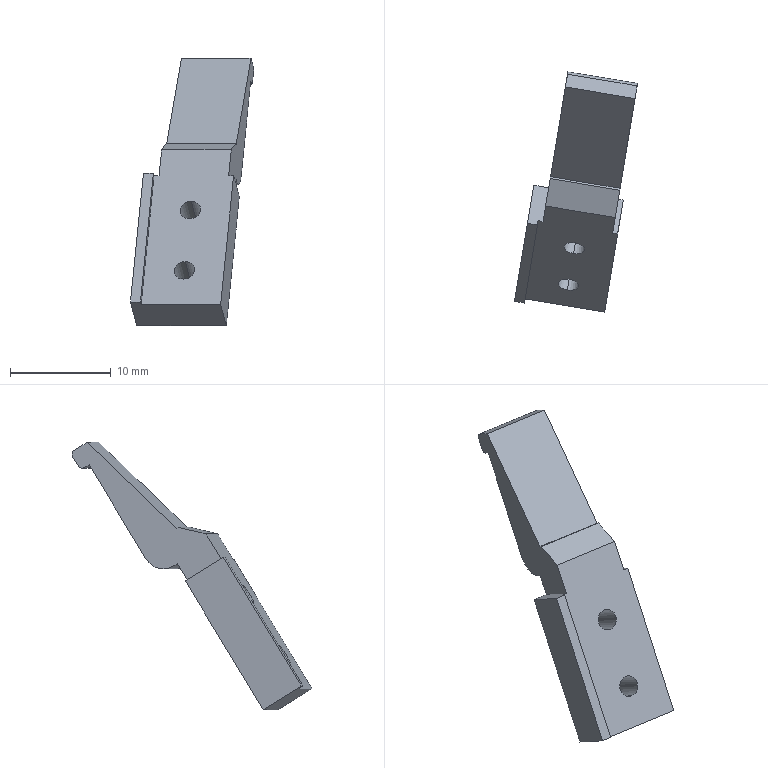Component | SolidWorks | 14AC-24-1-001-1 | 1 solid | 26 faces | box 12.21 x 23.8 x 26.53 mm | volume 925 mm3 | plane 19 | cylinder 7 | commonest cylinder face diameters 2.05 x4 1 x2 4 x1
build123d program:
from build123d import *

# Parameters (mm, degrees)
SKETCH1_W           = 9
SKETCH1_H           = 32
BOSS_EXTRUDE1_DEPTH = 7.45
SKETCH3_W           = 3.45
SKETCH3_H           = 17
CUT_EXTRUDE2_DEPTH  = 37.121
FILLET1_R           = 0.5
CUT_EXTRUDE6_DEPTH  = 37.121
SKETCH8_W           = 1
SKETCH8_H           = 13
CUT_EXTRUDE7_DEPTH  = 37.121
FILLET3_R           = 0.5
CHAMFER3_SIZE       = 2
FILLET5_R           = 2
M2_5_TAPPED_HOLE1_D = 2.05
SKETCH17_W          = 1
SKETCH17_H          = 18
BOSS_EXTRUDE2_DEPTH = 0.5
SKETCH18_W          = 3.461
SKETCH18_H          = 20.335
SKETCH18_H_2        = 25.647
CUT_EXTRUDE8_DEPTH  = 36.379


with BuildPart() as part:
    # Sketch1 → Boss-Extrude1 (new body)
    with BuildSketch(Plane.XY):
        with Locations((0, 18.179)):
            Rectangle(SKETCH1_W, SKETCH1_H)
    extrude(amount=BOSS_EXTRUDE1_DEPTH)

    # Sketch3 → Cut-Extrude2 (cut, through all)
    with BuildSketch(Plane(origin=(4.5, 0, 0), x_dir=(0, 0, -1), z_dir=(1, 0, 0))):
        with Locations((-1.725, 25.679)):
            Rectangle(SKETCH3_W, SKETCH3_H)
    extrude(amount=-CUT_EXTRUDE2_DEPTH, mode=Mode.SUBTRACT)

    # Fillet1
    fillet1_edges = [part.edges().sort_by_distance(p)[0] for p in [
        (0, 2.179, 0),
    ]]
    fillet(fillet1_edges, radius=FILLET1_R)

    # Sketch7 → Cut-Extrude6 (cut, through all)
    with BuildSketch(Plane(origin=(4.5, 0, 0), x_dir=(0, 0, -1), z_dir=(1, 0, 0))):
        Polygon((-7.45, 2.179), (-2, 2.179), (-5.215, 14.179), (-7.45, 14.179), align=None)
    extrude(amount=-CUT_EXTRUDE6_DEPTH, mode=Mode.SUBTRACT)

    # Sketch8 → Cut-Extrude7 (cut, through all)
    with BuildSketch(Plane(origin=(4.5, 0, 0), x_dir=(0, 0, -1), z_dir=(1, 0, 0))):
        with Locations((-0.5, 10.679)):
            Rectangle(SKETCH8_W, SKETCH8_H)
    extrude(amount=-CUT_EXTRUDE7_DEPTH, mode=Mode.SUBTRACT)

    # Fillet3
    fillet3_edges = [part.edges().sort_by_distance(p)[0] for p in [
        (0, 4.179, 0),
    ]]
    fillet(fillet3_edges, radius=FILLET3_R)

    # Chamfer3
    chamfer3_edges = [part.edges().sort_by_distance(p)[0] for p in [
        (0, 14.179, 7.45),
    ]]
    chamfer(chamfer3_edges, length=CHAMFER3_SIZE)

    # Fillet5
    fillet5_edges = [part.edges().sort_by_distance(p)[0] for p in [
        (0, 17.179, 1),
    ]]
    fillet(fillet5_edges, radius=FILLET5_R)

    # M2.5 Tapped Hole1 (through all)
    with Locations(Plane(origin=(0, 0, 3.45), x_dir=(-1, 0, 0), z_dir=(0, 0, -1))):
        with Locations((0.5, 23.179), (0.5, 30.179)):
            Hole(M2_5_TAPPED_HOLE1_D / 2)

    # Sketch17 → Boss-Extrude2 (add)
    with BuildSketch(Plane.XY.offset(7.45)):
        with Locations((4, 25.179)):
            Rectangle(SKETCH17_W, SKETCH17_H)
    extrude(amount=BOSS_EXTRUDE2_DEPTH)

    # Sketch18 → Cut-Extrude8 (cut, through all)
    with BuildSketch(Plane.XY.offset(7.95)):
        with Locations((-5.731, 9.012)):
            Rectangle(SKETCH18_W, SKETCH18_H)
        with Locations((4.731, 6.356)):
            Rectangle(SKETCH18_W, SKETCH18_H_2)
    extrude(amount=-CUT_EXTRUDE8_DEPTH, mode=Mode.SUBTRACT)


solid = part.part

# Placed as in the assembly
solid = solid.moved(Location((527.841, -215.325, 24.159), (58.173, -8.052, 175.031)))
STEP:
#1=COLOUR_RGB('',0.7922,0.8196,0.9333);
#2=FILL_AREA_STYLE_COLOUR('',#1);
#3=FILL_AREA_STYLE('',(#2));
#4=SURFACE_STYLE_FILL_AREA(#3);
#5=SURFACE_SIDE_STYLE('',(#4));
#6=SURFACE_STYLE_USAGE(.BOTH.,#5);
#7=PRESENTATION_STYLE_ASSIGNMENT((#6));
#8=CARTESIAN_POINT('',(20.685,-9.177,0.3604));
#9=VERTEX_POINT('',#8);
#10=CARTESIAN_POINT('',(20.678,-9.218,0.2916));
#11=VERTEX_POINT('',#10);
#12=CARTESIAN_POINT('',(20.681,-9.197,0.326));
#13=DIRECTION('',(0.1401,0.8413,-0.5222));
#14=DIRECTION('',(-0.08576,-0.5151,-0.8529));
#15=AXIS2_PLACEMENT_3D('',#12,#13,#14);
#16=CIRCLE('',#15,0.04035);
#17=EDGE_CURVE('',#9,#11,#16,.T.);
#18=ORIENTED_EDGE('',*,*,#17,.F.);
#19=CARTESIAN_POINT('',(20.707,-9.044,0.2782));
#20=VERTEX_POINT('',#19);
#21=CARTESIAN_POINT('',(20.707,-9.044,0.2782));
#22=DIRECTION('',(0.1401,0.8413,-0.5222));
#23=VECTOR('',#22,39.37);
#24=LINE('',#21,#23);
#25=EDGE_CURVE('',#9,#20,#24,.T.);
#26=ORIENTED_EDGE('',*,*,#25,.T.);
#27=CARTESIAN_POINT('',(20.7,-9.086,0.2094));
#28=VERTEX_POINT('',#27);
#29=CARTESIAN_POINT('',(20.703,-9.065,0.2438));
#30=DIRECTION('',(0.1401,0.8413,-0.5222));
#31=DIRECTION('',(-0.08576,-0.5151,-0.8529));
#32=AXIS2_PLACEMENT_3D('',#29,#30,#31);
#33=CIRCLE('',#32,0.04035);
#34=EDGE_CURVE('',#20,#28,#33,.T.);
#35=ORIENTED_EDGE('',*,*,#34,.T.);
#36=CARTESIAN_POINT('',(20.7,-9.086,0.2094));
#37=DIRECTION('',(0.1401,0.8413,-0.5222));
#38=VECTOR('',#37,39.37);
#39=LINE('',#36,#38);
#40=EDGE_CURVE('',#11,#28,#39,.T.);
#41=ORIENTED_EDGE('',*,*,#40,.F.);
#42=EDGE_LOOP('',(#18,#26,#35,#41));
#43=FACE_OUTER_BOUND('',#42,.T.);
#44=CARTESIAN_POINT('',(20.703,-9.065,0.2438));
#45=DIRECTION('',(0.1401,0.8413,-0.5222));
#46=DIRECTION('',(-0.08576,-0.5151,-0.8529));
#47=AXIS2_PLACEMENT_3D('',#44,#45,#46);
#48=CYLINDRICAL_SURFACE('',#47,0.04035);
#49=ADVANCED_FACE('',(#43),#48,.F.);
#50=CARTESIAN_POINT('',(20.661,-9.319,0.1254));
#51=VERTEX_POINT('',#50);
#52=CARTESIAN_POINT('',(20.654,-9.36,0.05656));
#53=VERTEX_POINT('',#52);
#54=CARTESIAN_POINT('',(20.658,-9.339,0.09097));
#55=DIRECTION('',(0.1401,0.8413,-0.5222));
#56=DIRECTION('',(-0.08576,-0.5151,-0.8529));
#57=AXIS2_PLACEMENT_3D('',#54,#55,#56);
#58=CIRCLE('',#57,0.04035);
#59=EDGE_CURVE('',#51,#53,#58,.T.);
#60=ORIENTED_EDGE('',*,*,#59,.F.);
#61=CARTESIAN_POINT('',(20.683,-9.186,0.04316));
#62=VERTEX_POINT('',#61);
#63=CARTESIAN_POINT('',(20.683,-9.186,0.04316));
#64=DIRECTION('',(0.1401,0.8413,-0.5222));
#65=VECTOR('',#64,39.37);
#66=LINE('',#63,#65);
#67=EDGE_CURVE('',#51,#62,#66,.T.);
#68=ORIENTED_EDGE('',*,*,#67,.T.);
#69=CARTESIAN_POINT('',(20.676,-9.228,-0.02567));
#70=VERTEX_POINT('',#69);
#71=CARTESIAN_POINT('',(20.68,-9.207,0.008744));
#72=DIRECTION('',(0.1401,0.8413,-0.5222));
#73=DIRECTION('',(-0.08576,-0.5151,-0.8529));
#74=AXIS2_PLACEMENT_3D('',#71,#72,#73);
#75=CIRCLE('',#74,0.04035);
#76=EDGE_CURVE('',#62,#70,#75,.T.);
#77=ORIENTED_EDGE('',*,*,#76,.T.);
#78=CARTESIAN_POINT('',(20.676,-9.228,-0.02567));
#79=DIRECTION('',(0.1401,0.8413,-0.5222));
#80=VECTOR('',#79,39.37);
#81=LINE('',#78,#80);
#82=EDGE_CURVE('',#53,#70,#81,.T.);
#83=ORIENTED_EDGE('',*,*,#82,.F.);
#84=EDGE_LOOP('',(#60,#68,#77,#83));
#85=FACE_OUTER_BOUND('',#84,.T.);
#86=CARTESIAN_POINT('',(20.68,-9.207,0.008744));
#87=DIRECTION('',(0.1401,0.8413,-0.5222));
#88=DIRECTION('',(-0.08576,-0.5151,-0.8529));
#89=AXIS2_PLACEMENT_3D('',#86,#87,#88);
#90=CYLINDRICAL_SURFACE('',#89,0.04035);
#91=ADVANCED_FACE('',(#85),#90,.F.);
#92=CARTESIAN_POINT('',(20.658,-9.339,0.09097));
#93=DIRECTION('',(0.1401,0.8413,-0.5222));
#94=DIRECTION('',(-0.08576,-0.5151,-0.8529));
#95=AXIS2_PLACEMENT_3D('',#92,#93,#94);
#96=CIRCLE('',#95,0.04035);
#97=EDGE_CURVE('',#53,#51,#96,.T.);
#98=ORIENTED_EDGE('',*,*,#97,.T.);
#99=ORIENTED_EDGE('',*,*,#59,.T.);
#100=EDGE_LOOP('',(#98,#99));
#101=FACE_BOUND('',#100,.T.);
#102=CARTESIAN_POINT('',(20.681,-9.197,0.326));
#103=DIRECTION('',(0.1401,0.8413,-0.5222));
#104=DIRECTION('',(-0.08576,-0.5151,-0.8529));
#105=AXIS2_PLACEMENT_3D('',#102,#103,#104);
#106=CIRCLE('',#105,0.04035);
#107=EDGE_CURVE('',#11,#9,#106,.T.);
#108=ORIENTED_EDGE('',*,*,#107,.T.);
#109=ORIENTED_EDGE('',*,*,#17,.T.);
#110=EDGE_LOOP('',(#108,#109));
#111=FACE_BOUND('',#110,.T.);
#112=CARTESIAN_POINT('',(20.841,-9.078,0.561));
#113=VERTEX_POINT('',#112);
#114=CARTESIAN_POINT('',(20.569,-9.033,0.561));
#115=VERTEX_POINT('',#114);
#116=CARTESIAN_POINT('',(20.86,-9.081,0.561));
#117=DIRECTION('',(-0.9864,0.1642,-0.));
#118=VECTOR('',#117,39.37);
#119=LINE('',#116,#118);
#120=EDGE_CURVE('',#113,#115,#119,.T.);
#121=ORIENTED_EDGE('',*,*,#120,.T.);
#122=CARTESIAN_POINT('',(20.559,-9.094,0.4603));
#123=VERTEX_POINT('',#122);
#124=CARTESIAN_POINT('',(20.508,-9.398,-0.04333));
#125=DIRECTION('',(-0.08576,-0.5151,-0.8529));
#126=VECTOR('',#125,39.37);
#127=LINE('',#124,#126);
#128=EDGE_CURVE('',#115,#123,#127,.T.);
#129=ORIENTED_EDGE('',*,*,#128,.T.);
#130=CARTESIAN_POINT('',(20.539,-9.09,0.4603));
#131=VERTEX_POINT('',#130);
#132=CARTESIAN_POINT('',(20.85,-9.142,0.4603));
#133=DIRECTION('',(-0.9864,0.1642,-0.));
#134=VECTOR('',#133,39.37);
#135=LINE('',#132,#134);
#136=EDGE_CURVE('',#123,#131,#135,.T.);
#137=ORIENTED_EDGE('',*,*,#136,.T.);
#138=CARTESIAN_POINT('',(20.489,-9.395,-0.04333));
#139=VERTEX_POINT('',#138);
#140=CARTESIAN_POINT('',(20.55,-9.03,0.561));
#141=DIRECTION('',(0.08576,0.5151,0.8529));
#142=VECTOR('',#141,39.37);
#143=LINE('',#140,#142);
#144=EDGE_CURVE('',#139,#131,#143,.T.);
#145=ORIENTED_EDGE('',*,*,#144,.F.);
#146=CARTESIAN_POINT('',(20.799,-9.446,-0.04333));
#147=VERTEX_POINT('',#146);
#148=CARTESIAN_POINT('',(20.799,-9.446,-0.04333));
#149=DIRECTION('',(0.9864,-0.1642,0.));
#150=VECTOR('',#149,39.37);
#151=LINE('',#148,#150);
#152=EDGE_CURVE('',#139,#147,#151,.T.);
#153=ORIENTED_EDGE('',*,*,#152,.T.);
#154=CARTESIAN_POINT('',(20.85,-9.142,0.4603));
#155=VERTEX_POINT('',#154);
#156=CARTESIAN_POINT('',(20.907,-8.797,1.031));
#157=DIRECTION('',(0.08576,0.5151,0.8529));
#158=VECTOR('',#157,39.37);
#159=LINE('',#156,#158);
#160=EDGE_CURVE('',#147,#155,#159,.T.);
#161=ORIENTED_EDGE('',*,*,#160,.T.);
#162=CARTESIAN_POINT('',(20.831,-9.139,0.4603));
#163=VERTEX_POINT('',#162);
#164=CARTESIAN_POINT('',(20.85,-9.142,0.4603));
#165=DIRECTION('',(-0.9864,0.1642,-0.));
#166=VECTOR('',#165,39.37);
#167=LINE('',#164,#166);
#168=EDGE_CURVE('',#155,#163,#167,.T.);
#169=ORIENTED_EDGE('',*,*,#168,.T.);
#170=CARTESIAN_POINT('',(20.78,-9.443,-0.04333));
#171=DIRECTION('',(0.08576,0.5151,0.8529));
#172=VECTOR('',#171,39.37);
#173=LINE('',#170,#172);
#174=EDGE_CURVE('',#163,#113,#173,.T.);
#175=ORIENTED_EDGE('',*,*,#174,.T.);
#176=EDGE_LOOP('',(#121,#129,#137,#145,#153,#161,#169,#175));
#177=FACE_OUTER_BOUND('',#176,.T.);
#178=CARTESIAN_POINT('',(20.799,-9.446,-0.04333));
#179=DIRECTION('',(0.1401,0.8413,-0.5222));
#180=DIRECTION('',(0.9864,-0.1642,0.));
#181=AXIS2_PLACEMENT_3D('',#178,#179,#180);
#182=PLANE('',#181);
#183=ADVANCED_FACE('',(#101,#111,#177),#182,.F.);
#184=CARTESIAN_POINT('',(20.821,-9.314,-0.1256));
#185=VERTEX_POINT('',#184);
#186=CARTESIAN_POINT('',(20.872,-9.01,0.3781));
#187=VERTEX_POINT('',#186);
#188=CARTESIAN_POINT('',(20.821,-9.314,-0.1256));
#189=DIRECTION('',(0.08576,0.5151,0.8529));
#190=VECTOR('',#189,39.37);
#191=LINE('',#188,#190);
#192=EDGE_CURVE('',#185,#187,#191,.T.);
#193=ORIENTED_EDGE('',*,*,#192,.T.);
#194=CARTESIAN_POINT('',(20.85,-9.142,0.4603));
#195=DIRECTION('',(-0.1401,-0.8413,0.5222));
#196=VECTOR('',#195,39.37);
#197=LINE('',#194,#196);
#198=EDGE_CURVE('',#187,#155,#197,.T.);
#199=ORIENTED_EDGE('',*,*,#198,.T.);
#200=ORIENTED_EDGE('',*,*,#160,.F.);
#201=CARTESIAN_POINT('',(20.799,-9.446,-0.04333));
#202=DIRECTION('',(0.1401,0.8413,-0.5222));
#203=VECTOR('',#202,39.37);
#204=LINE('',#201,#203);
#205=EDGE_CURVE('',#147,#185,#204,.T.);
#206=ORIENTED_EDGE('',*,*,#205,.T.);
#207=EDGE_LOOP('',(#193,#199,#200,#206));
#208=FACE_OUTER_BOUND('',#207,.T.);
#209=CARTESIAN_POINT('',(20.907,-8.797,1.031));
#210=DIRECTION('',(-0.9864,0.1642,-0.));
#211=DIRECTION('',(0.1401,0.8413,-0.5222));
#212=AXIS2_PLACEMENT_3D('',#209,#210,#211);
#213=PLANE('',#212);
#214=ADVANCED_FACE('',(#208),#213,.F.);
#215=CARTESIAN_POINT('',(20.926,-8.564,0.8883));
#216=VERTEX_POINT('',#215);
#217=CARTESIAN_POINT('',(20.655,-8.519,0.8883));
#218=VERTEX_POINT('',#217);
#219=CARTESIAN_POINT('',(20.596,-8.509,0.8883));
#220=DIRECTION('',(-0.9864,0.1642,-0.));
#221=VECTOR('',#220,39.37);
#222=LINE('',#219,#221);
#223=EDGE_CURVE('',#216,#218,#222,.T.);
#224=ORIENTED_EDGE('',*,*,#223,.T.);
#225=CARTESIAN_POINT('',(20.646,-8.568,0.9191));
#226=VERTEX_POINT('',#225);
#227=CARTESIAN_POINT('',(20.616,-8.749,1.031));
#228=DIRECTION('',(-0.1401,-0.8413,0.5222));
#229=VECTOR('',#228,39.37);
#230=LINE('',#227,#229);
#231=EDGE_CURVE('',#218,#226,#230,.T.);
#232=ORIENTED_EDGE('',*,*,#231,.T.);
#233=CARTESIAN_POINT('',(20.918,-8.614,0.9191));
#234=VERTEX_POINT('',#233);
#235=CARTESIAN_POINT('',(20.938,-8.617,0.9191));
#236=DIRECTION('',(-0.9864,0.1642,-0.));
#237=VECTOR('',#236,39.37);
#238=LINE('',#235,#237);
#239=EDGE_CURVE('',#234,#226,#238,.T.);
#240=ORIENTED_EDGE('',*,*,#239,.F.);
#241=CARTESIAN_POINT('',(20.888,-8.794,1.031));
#242=DIRECTION('',(0.1401,0.8413,-0.5222));
#243=VECTOR('',#242,39.37);
#244=LINE('',#241,#243);
#245=EDGE_CURVE('',#234,#216,#244,.T.);
#246=ORIENTED_EDGE('',*,*,#245,.T.);
#247=EDGE_LOOP('',(#224,#232,#240,#246));
#248=FACE_OUTER_BOUND('',#247,.T.);
#249=CARTESIAN_POINT('',(20.907,-8.797,1.031));
#250=DIRECTION('',(-0.08576,-0.5151,-0.8529));
#251=DIRECTION('',(-0.1401,-0.8413,0.5222));
#252=AXIS2_PLACEMENT_3D('',#249,#250,#251);
#253=PLANE('',#252);
#254=ADVANCED_FACE('',(#248),#253,.F.);
#255=CARTESIAN_POINT('',(20.498,-9.1,0.4706));
#256=VERTEX_POINT('',#255);
#257=CARTESIAN_POINT('',(20.447,-9.405,-0.03305));
#258=VERTEX_POINT('',#257);
#259=CARTESIAN_POINT('',(20.508,-9.04,0.5713));
#260=DIRECTION('',(-0.08576,-0.5151,-0.8529));
#261=VECTOR('',#260,39.37);
#262=LINE('',#259,#261);
#263=EDGE_CURVE('',#256,#258,#262,.T.);
#264=ORIENTED_EDGE('',*,*,#263,.F.);
#265=CARTESIAN_POINT('',(20.523,-8.951,0.3781));
#266=VERTEX_POINT('',#265);
#267=CARTESIAN_POINT('',(20.501,-9.084,0.4603));
#268=DIRECTION('',(0.1401,0.8413,-0.5222));
#269=VECTOR('',#268,39.37);
#270=LINE('',#267,#269);
#271=EDGE_CURVE('',#256,#266,#270,.T.);
#272=ORIENTED_EDGE('',*,*,#271,.T.);
#273=CARTESIAN_POINT('',(20.472,-9.256,-0.1256));
#274=VERTEX_POINT('',#273);
#275=CARTESIAN_POINT('',(20.472,-9.256,-0.1256));
#276=DIRECTION('',(0.08576,0.5151,0.8529));
#277=VECTOR('',#276,39.37);
#278=LINE('',#275,#277);
#279=EDGE_CURVE('',#274,#266,#278,.T.);
#280=ORIENTED_EDGE('',*,*,#279,.F.);
#281=CARTESIAN_POINT('',(20.45,-9.388,-0.04333));
#282=DIRECTION('',(0.1401,0.8413,-0.5222));
#283=VECTOR('',#282,39.37);
#284=LINE('',#281,#283);
#285=EDGE_CURVE('',#258,#274,#284,.T.);
#286=ORIENTED_EDGE('',*,*,#285,.F.);
#287=EDGE_LOOP('',(#264,#272,#280,#286));
#288=FACE_OUTER_BOUND('',#287,.T.);
#289=CARTESIAN_POINT('',(20.558,-8.739,1.031));
#290=DIRECTION('',(0.9864,-0.1642,0.));
#291=DIRECTION('',(-0.1401,-0.8413,0.5222));
#292=AXIS2_PLACEMENT_3D('',#289,#290,#291);
#293=PLANE('',#292);
#294=ADVANCED_FACE('',(#288),#293,.F.);
#295=ORIENTED_EDGE('',*,*,#285,.T.);
#296=CARTESIAN_POINT('',(20.821,-9.314,-0.1256));
#297=DIRECTION('',(-0.9864,0.1642,-0.));
#298=VECTOR('',#297,39.37);
#299=LINE('',#296,#298);
#300=EDGE_CURVE('',#185,#274,#299,.T.);
#301=ORIENTED_EDGE('',*,*,#300,.F.);
#302=ORIENTED_EDGE('',*,*,#205,.F.);
#303=ORIENTED_EDGE('',*,*,#152,.F.);
#304=CARTESIAN_POINT('',(20.486,-9.411,-0.03305));
#305=VERTEX_POINT('',#304);
#306=CARTESIAN_POINT('',(20.486,-9.411,-0.03305));
#307=DIRECTION('',(0.1401,0.8413,-0.5222));
#308=VECTOR('',#307,39.37);
#309=LINE('',#306,#308);
#310=EDGE_CURVE('',#305,#139,#309,.T.);
#311=ORIENTED_EDGE('',*,*,#310,.F.);
#312=CARTESIAN_POINT('',(20.447,-9.405,-0.03305));
#313=DIRECTION('',(0.9864,-0.1642,0.));
#314=VECTOR('',#313,39.37);
#315=LINE('',#312,#314);
#316=EDGE_CURVE('',#258,#305,#315,.T.);
#317=ORIENTED_EDGE('',*,*,#316,.F.);
#318=EDGE_LOOP('',(#295,#301,#302,#303,#311,#317));
#319=FACE_OUTER_BOUND('',#318,.T.);
#320=CARTESIAN_POINT('',(20.799,-9.446,-0.04333));
#321=DIRECTION('',(0.08576,0.5151,0.8529));
#322=DIRECTION('',(0.1401,0.8413,-0.5222));
#323=AXIS2_PLACEMENT_3D('',#320,#321,#322);
#324=PLANE('',#323);
#325=ADVANCED_FACE('',(#319),#324,.F.);
#326=CARTESIAN_POINT('',(20.652,-8.533,0.8276));
#327=VERTEX_POINT('',#326);
#328=CARTESIAN_POINT('',(20.656,-8.512,0.8612));
#329=VERTEX_POINT('',#328);
#330=CARTESIAN_POINT('',(20.6,-8.847,0.3072));
#331=DIRECTION('',(0.08576,0.5151,0.8529));
#332=VECTOR('',#331,39.37);
#333=LINE('',#330,#332);
#334=EDGE_CURVE('',#327,#329,#333,.T.);
#335=ORIENTED_EDGE('',*,*,#334,.T.);
#336=CARTESIAN_POINT('',(20.927,-8.558,0.8612));
#337=VERTEX_POINT('',#336);
#338=CARTESIAN_POINT('',(20.947,-8.561,0.8612));
#339=DIRECTION('',(0.9864,-0.1642,0.));
#340=VECTOR('',#339,39.37);
#341=LINE('',#338,#340);
#342=EDGE_CURVE('',#329,#337,#341,.T.);
#343=ORIENTED_EDGE('',*,*,#342,.T.);
#344=CARTESIAN_POINT('',(20.924,-8.578,0.8276));
#345=VERTEX_POINT('',#344);
#346=CARTESIAN_POINT('',(20.872,-8.892,0.3072));
#347=DIRECTION('',(-0.08576,-0.5151,-0.8529));
#348=VECTOR('',#347,39.37);
#349=LINE('',#346,#348);
#350=EDGE_CURVE('',#337,#345,#349,.T.);
#351=ORIENTED_EDGE('',*,*,#350,.T.);
#352=CARTESIAN_POINT('',(20.594,-8.523,0.8276));
#353=DIRECTION('',(-0.9864,0.1642,-0.));
#354=VECTOR('',#353,39.37);
#355=LINE('',#352,#354);
#356=EDGE_CURVE('',#345,#327,#355,.T.);
#357=ORIENTED_EDGE('',*,*,#356,.T.);
#358=EDGE_LOOP('',(#335,#343,#351,#357));
#359=FACE_OUTER_BOUND('',#358,.T.);
#360=CARTESIAN_POINT('',(20.841,-9.2,-0.1965));
#361=DIRECTION('',(0.1401,0.8413,-0.5222));
#362=DIRECTION('',(0.9864,-0.1642,0.));
#363=AXIS2_PLACEMENT_3D('',#360,#361,#362);
#364=PLANE('',#363);
#365=ADVANCED_FACE('',(#359),#364,.T.);
#366=CARTESIAN_POINT('',(20.859,-8.966,0.4452));
#367=VERTEX_POINT('',#366);
#368=CARTESIAN_POINT('',(20.588,-8.921,0.4452));
#369=VERTEX_POINT('',#368);
#370=CARTESIAN_POINT('',(20.879,-8.969,0.4452));
#371=DIRECTION('',(-0.9864,0.1642,-0.));
#372=VECTOR('',#371,39.37);
#373=LINE('',#370,#372);
#374=EDGE_CURVE('',#367,#369,#373,.T.);
#375=ORIENTED_EDGE('',*,*,#374,.T.);
#376=CARTESIAN_POINT('',(20.59,-8.906,0.436));
#377=VERTEX_POINT('',#376);
#378=CARTESIAN_POINT('',(20.588,-8.921,0.4452));
#379=DIRECTION('',(0.1401,0.8413,-0.5222));
#380=VECTOR('',#379,39.37);
#381=LINE('',#378,#380);
#382=EDGE_CURVE('',#369,#377,#381,.T.);
#383=ORIENTED_EDGE('',*,*,#382,.T.);
#384=CARTESIAN_POINT('',(20.862,-8.951,0.436));
#385=VERTEX_POINT('',#384);
#386=CARTESIAN_POINT('',(20.881,-8.954,0.436));
#387=DIRECTION('',(0.9864,-0.1642,0.));
#388=VECTOR('',#387,39.37);
#389=LINE('',#386,#388);
#390=EDGE_CURVE('',#377,#385,#389,.T.);
#391=ORIENTED_EDGE('',*,*,#390,.T.);
#392=CARTESIAN_POINT('',(20.859,-8.966,0.4452));
#393=DIRECTION('',(-0.1401,-0.8413,0.5222));
#394=VECTOR('',#393,39.37);
#395=LINE('',#392,#394);
#396=EDGE_CURVE('',#385,#367,#395,.T.);
#397=ORIENTED_EDGE('',*,*,#396,.T.);
#398=EDGE_LOOP('',(#375,#383,#391,#397));
#399=FACE_OUTER_BOUND('',#398,.T.);
#400=CARTESIAN_POINT('',(20.879,-8.969,0.4452));
#401=DIRECTION('',(0.08576,0.5151,0.8529));
#402=DIRECTION('',(0.1401,0.8413,-0.5222));
#403=AXIS2_PLACEMENT_3D('',#400,#401,#402);
#404=PLANE('',#403);
#405=ADVANCED_FACE('',(#399),#404,.F.);
#406=CARTESIAN_POINT('',(20.703,-9.065,0.2438));
#407=DIRECTION('',(0.1401,0.8413,-0.5222));
#408=DIRECTION('',(-0.08576,-0.5151,-0.8529));
#409=AXIS2_PLACEMENT_3D('',#406,#407,#408);
#410=CIRCLE('',#409,0.04035);
#411=EDGE_CURVE('',#28,#20,#410,.T.);
#412=ORIENTED_EDGE('',*,*,#411,.F.);
#413=ORIENTED_EDGE('',*,*,#34,.F.);
#414=EDGE_LOOP('',(#412,#413));
#415=FACE_BOUND('',#414,.T.);
#416=CARTESIAN_POINT('',(20.68,-9.207,0.008744));
#417=DIRECTION('',(0.1401,0.8413,-0.5222));
#418=DIRECTION('',(-0.08576,-0.5151,-0.8529));
#419=AXIS2_PLACEMENT_3D('',#416,#417,#418);
#420=CIRCLE('',#419,0.04035);
#421=EDGE_CURVE('',#70,#62,#420,.T.);
#422=ORIENTED_EDGE('',*,*,#421,.F.);
#423=ORIENTED_EDGE('',*,*,#76,.F.);
#424=EDGE_LOOP('',(#422,#423));
#425=FACE_BOUND('',#424,.T.);
#426=CARTESIAN_POINT('',(20.581,-8.961,0.3781));
#427=VERTEX_POINT('',#426);
#428=CARTESIAN_POINT('',(20.872,-9.01,0.3781));
#429=DIRECTION('',(0.9864,-0.1642,0.));
#430=VECTOR('',#429,39.37);
#431=LINE('',#428,#430);
#432=EDGE_CURVE('',#266,#427,#431,.T.);
#433=ORIENTED_EDGE('',*,*,#432,.T.);
#434=CARTESIAN_POINT('',(20.53,-9.265,-0.1256));
#435=DIRECTION('',(0.08576,0.5151,0.8529));
#436=VECTOR('',#435,39.37);
#437=LINE('',#434,#436);
#438=EDGE_CURVE('',#427,#369,#437,.T.);
#439=ORIENTED_EDGE('',*,*,#438,.T.);
#440=ORIENTED_EDGE('',*,*,#374,.F.);
#441=CARTESIAN_POINT('',(20.853,-9.006,0.3781));
#442=VERTEX_POINT('',#441);
#443=CARTESIAN_POINT('',(20.802,-9.311,-0.1256));
#444=DIRECTION('',(-0.08576,-0.5151,-0.8529));
#445=VECTOR('',#444,39.37);
#446=LINE('',#443,#445);
#447=EDGE_CURVE('',#367,#442,#446,.T.);
#448=ORIENTED_EDGE('',*,*,#447,.T.);
#449=CARTESIAN_POINT('',(20.872,-9.01,0.3781));
#450=DIRECTION('',(0.9864,-0.1642,0.));
#451=VECTOR('',#450,39.37);
#452=LINE('',#449,#451);
#453=EDGE_CURVE('',#442,#187,#452,.T.);
#454=ORIENTED_EDGE('',*,*,#453,.T.);
#455=ORIENTED_EDGE('',*,*,#192,.F.);
#456=ORIENTED_EDGE('',*,*,#300,.T.);
#457=ORIENTED_EDGE('',*,*,#279,.T.);
#458=EDGE_LOOP('',(#433,#439,#440,#448,#454,#455,#456,#457));
#459=FACE_OUTER_BOUND('',#458,.T.);
#460=CARTESIAN_POINT('',(20.821,-9.314,-0.1256));
#461=DIRECTION('',(-0.1401,-0.8413,0.5222));
#462=DIRECTION('',(0.08576,0.5151,0.8529));
#463=AXIS2_PLACEMENT_3D('',#460,#461,#462);
#464=PLANE('',#463);
#465=ADVANCED_FACE('',(#415,#425,#459),#464,.F.);
#466=CARTESIAN_POINT('',(20.653,-8.529,0.8715));
#467=DIRECTION('',(-0.9864,0.1642,-0.));
#468=DIRECTION('',(0.08576,0.5151,0.8529));
#469=AXIS2_PLACEMENT_3D('',#466,#467,#468);
#470=CIRCLE('',#469,0.01969);
#471=EDGE_CURVE('',#218,#329,#470,.T.);
#472=ORIENTED_EDGE('',*,*,#471,.F.);
#473=ORIENTED_EDGE('',*,*,#223,.F.);
#474=CARTESIAN_POINT('',(20.925,-8.574,0.8715));
#475=DIRECTION('',(0.9864,-0.1642,0.));
#476=DIRECTION('',(-0.08576,-0.5151,-0.8529));
#477=AXIS2_PLACEMENT_3D('',#474,#475,#476);
#478=CIRCLE('',#477,0.01969);
#479=EDGE_CURVE('',#337,#216,#478,.T.);
#480=ORIENTED_EDGE('',*,*,#479,.F.);
#481=ORIENTED_EDGE('',*,*,#342,.F.);
#482=EDGE_LOOP('',(#472,#473,#480,#481));
#483=FACE_OUTER_BOUND('',#482,.T.);
#484=CARTESIAN_POINT('',(20.944,-8.577,0.8715));
#485=DIRECTION('',(0.9864,-0.1642,0.));
#486=DIRECTION('',(-0.1401,-0.8413,0.5222));
#487=AXIS2_PLACEMENT_3D('',#484,#485,#486);
#488=CYLINDRICAL_SURFACE('',#487,0.01969);
#489=ADVANCED_FACE('',(#483),#488,.T.);
#490=CARTESIAN_POINT('',(20.86,-8.963,0.5823));
#491=VERTEX_POINT('',#490);
#492=CARTESIAN_POINT('',(20.588,-8.918,0.5823));
#493=VERTEX_POINT('',#492);
#494=CARTESIAN_POINT('',(20.879,-8.967,0.5823));
#495=DIRECTION('',(-0.9864,0.1642,-0.));
#496=VECTOR('',#495,39.37);
#497=LINE('',#494,#496);
#498=EDGE_CURVE('',#491,#493,#497,.T.);
#499=ORIENTED_EDGE('',*,*,#498,.T.);
#500=CARTESIAN_POINT('',(20.587,-8.926,0.5871));
#501=VERTEX_POINT('',#500);
#502=CARTESIAN_POINT('',(20.588,-8.918,0.5823));
#503=DIRECTION('',(-0.1401,-0.8413,0.5222));
#504=VECTOR('',#503,39.37);
#505=LINE('',#502,#504);
#506=EDGE_CURVE('',#493,#501,#505,.T.);
#507=ORIENTED_EDGE('',*,*,#506,.T.);
#508=CARTESIAN_POINT('',(20.859,-8.971,0.5871));
#509=VERTEX_POINT('',#508);
#510=CARTESIAN_POINT('',(20.878,-8.975,0.5871));
#511=DIRECTION('',(0.9864,-0.1642,0.));
#512=VECTOR('',#511,39.37);
#513=LINE('',#510,#512);
#514=EDGE_CURVE('',#501,#509,#513,.T.);
#515=ORIENTED_EDGE('',*,*,#514,.T.);
#516=CARTESIAN_POINT('',(20.86,-8.963,0.5823));
#517=DIRECTION('',(0.1401,0.8413,-0.5222));
#518=VECTOR('',#517,39.37);
#519=LINE('',#516,#518);
#520=EDGE_CURVE('',#509,#491,#519,.T.);
#521=ORIENTED_EDGE('',*,*,#520,.T.);
#522=EDGE_LOOP('',(#499,#507,#515,#521));
#523=FACE_OUTER_BOUND('',#522,.T.);
#524=CARTESIAN_POINT('',(20.879,-8.967,0.5823));
#525=DIRECTION('',(-0.08576,-0.5151,-0.8529));
#526=DIRECTION('',(-0.1401,-0.8413,0.5222));
#527=AXIS2_PLACEMENT_3D('',#524,#525,#526);
#528=PLANE('',#527);
#529=ADVANCED_FACE('',(#523),#528,.F.);
#530=ORIENTED_EDGE('',*,*,#239,.T.);
#531=CARTESIAN_POINT('',(20.646,-8.568,0.9191));
#532=DIRECTION('',(-0.1191,-0.7152,-0.6886));
#533=VECTOR('',#532,39.37);
#534=LINE('',#531,#533);
#535=EDGE_CURVE('',#226,#493,#534,.T.);
#536=ORIENTED_EDGE('',*,*,#535,.T.);
#537=ORIENTED_EDGE('',*,*,#498,.F.);
#538=CARTESIAN_POINT('',(20.918,-8.614,0.9191));
#539=DIRECTION('',(0.1191,0.7152,0.6886));
#540=VECTOR('',#539,39.37);
#541=LINE('',#538,#540);
#542=EDGE_CURVE('',#491,#234,#541,.T.);
#543=ORIENTED_EDGE('',*,*,#542,.T.);
#544=EDGE_LOOP('',(#530,#536,#537,#543));
#545=FACE_OUTER_BOUND('',#544,.T.);
#546=CARTESIAN_POINT('',(20.938,-8.617,0.9191));
#547=DIRECTION('',(0.1131,0.6793,-0.7251));
#548=DIRECTION('',(-0.1191,-0.7152,-0.6886));
#549=AXIS2_PLACEMENT_3D('',#546,#547,#548);
#550=PLANE('',#549);
#551=ADVANCED_FACE('',(#545),#550,.F.);
#552=CARTESIAN_POINT('',(20.917,-8.621,0.8314));
#553=VERTEX_POINT('',#552);
#554=CARTESIAN_POINT('',(20.645,-8.576,0.8314));
#555=VERTEX_POINT('',#554);
#556=CARTESIAN_POINT('',(20.936,-8.624,0.8314));
#557=DIRECTION('',(-0.9864,0.1642,-0.));
#558=VECTOR('',#557,39.37);
#559=LINE('',#556,#558);
#560=EDGE_CURVE('',#553,#555,#559,.T.);
#561=ORIENTED_EDGE('',*,*,#560,.T.);
#562=CARTESIAN_POINT('',(20.648,-8.559,0.8211));
#563=VERTEX_POINT('',#562);
#564=CARTESIAN_POINT('',(20.651,-8.543,0.8108));
#565=DIRECTION('',(0.1401,0.8413,-0.5222));
#566=VECTOR('',#565,39.37);
#567=LINE('',#564,#566);
#568=EDGE_CURVE('',#555,#563,#567,.T.);
#569=ORIENTED_EDGE('',*,*,#568,.T.);
#570=CARTESIAN_POINT('',(20.92,-8.605,0.8211));
#571=VERTEX_POINT('',#570);
#572=CARTESIAN_POINT('',(20.939,-8.608,0.8211));
#573=DIRECTION('',(0.9864,-0.1642,0.));
#574=VECTOR('',#573,39.37);
#575=LINE('',#572,#574);
#576=EDGE_CURVE('',#563,#571,#575,.T.);
#577=ORIENTED_EDGE('',*,*,#576,.T.);
#578=CARTESIAN_POINT('',(20.922,-8.588,0.8108));
#579=DIRECTION('',(-0.1401,-0.8413,0.5222));
#580=VECTOR('',#579,39.37);
#581=LINE('',#578,#580);
#582=EDGE_CURVE('',#571,#553,#581,.T.);
#583=ORIENTED_EDGE('',*,*,#582,.T.);
#584=EDGE_LOOP('',(#561,#569,#577,#583));
#585=FACE_OUTER_BOUND('',#584,.T.);
#586=CARTESIAN_POINT('',(20.942,-8.591,0.8108));
#587=DIRECTION('',(0.08576,0.5151,0.8529));
#588=DIRECTION('',(0.1401,0.8413,-0.5222));
#589=AXIS2_PLACEMENT_3D('',#586,#587,#588);
#590=PLANE('',#589);
#591=ADVANCED_FACE('',(#585),#590,.F.);
#592=CARTESIAN_POINT('',(20.88,-8.844,0.462));
#593=VERTEX_POINT('',#592);
#594=CARTESIAN_POINT('',(20.608,-8.799,0.462));
#595=VERTEX_POINT('',#594);
#596=CARTESIAN_POINT('',(20.899,-8.847,0.462));
#597=DIRECTION('',(-0.9864,0.1642,-0.));
#598=VECTOR('',#597,39.37);
#599=LINE('',#596,#598);
#600=EDGE_CURVE('',#593,#595,#599,.T.);
#601=ORIENTED_EDGE('',*,*,#600,.T.);
#602=CARTESIAN_POINT('',(20.601,-8.839,0.3949));
#603=DIRECTION('',(0.08576,0.5151,0.8529));
#604=VECTOR('',#603,39.37);
#605=LINE('',#602,#604);
#606=EDGE_CURVE('',#595,#555,#605,.T.);
#607=ORIENTED_EDGE('',*,*,#606,.T.);
#608=ORIENTED_EDGE('',*,*,#560,.F.);
#609=CARTESIAN_POINT('',(20.873,-8.885,0.3949));
#610=DIRECTION('',(-0.08576,-0.5151,-0.8529));
#611=VECTOR('',#610,39.37);
#612=LINE('',#609,#611);
#613=EDGE_CURVE('',#553,#593,#612,.T.);
#614=ORIENTED_EDGE('',*,*,#613,.T.);
#615=EDGE_LOOP('',(#601,#607,#608,#614));
#616=FACE_OUTER_BOUND('',#615,.T.);
#617=CARTESIAN_POINT('',(20.892,-8.888,0.3949));
#618=DIRECTION('',(-0.1401,-0.8413,0.5222));
#619=DIRECTION('',(0.08576,0.5151,0.8529));
#620=AXIS2_PLACEMENT_3D('',#617,#618,#619);
#621=PLANE('',#620);
#622=ADVANCED_FACE('',(#616),#621,.F.);
#623=CARTESIAN_POINT('',(20.649,-8.549,0.8379));
#624=DIRECTION('',(-0.9864,0.1642,-0.));
#625=DIRECTION('',(0.08576,0.5151,0.8529));
#626=AXIS2_PLACEMENT_3D('',#623,#624,#625);
#627=CIRCLE('',#626,0.01969);
#628=EDGE_CURVE('',#327,#563,#627,.T.);
#629=ORIENTED_EDGE('',*,*,#628,.F.);
#630=ORIENTED_EDGE('',*,*,#356,.F.);
#631=CARTESIAN_POINT('',(20.921,-8.594,0.8379));
#632=DIRECTION('',(0.9864,-0.1642,0.));
#633=DIRECTION('',(-0.08576,-0.5151,-0.8529));
#634=AXIS2_PLACEMENT_3D('',#631,#632,#633);
#635=CIRCLE('',#634,0.01969);
#636=EDGE_CURVE('',#571,#345,#635,.T.);
#637=ORIENTED_EDGE('',*,*,#636,.F.);
#638=ORIENTED_EDGE('',*,*,#576,.F.);
#639=EDGE_LOOP('',(#629,#630,#637,#638));
#640=FACE_OUTER_BOUND('',#639,.T.);
#641=CARTESIAN_POINT('',(20.941,-8.598,0.8379));
#642=DIRECTION('',(0.9864,-0.1642,0.));
#643=DIRECTION('',(-0.1401,-0.8413,0.5222));
#644=AXIS2_PLACEMENT_3D('',#641,#642,#643);
#645=CYLINDRICAL_SURFACE('',#644,0.01969);
#646=ADVANCED_FACE('',(#640),#645,.T.);
#647=CARTESIAN_POINT('',(20.569,-9.033,0.561));
#648=DIRECTION('',(0.1597,0.9591,0.2338));
#649=VECTOR('',#648,39.37);
#650=LINE('',#647,#649);
#651=EDGE_CURVE('',#115,#501,#650,.T.);
#652=ORIENTED_EDGE('',*,*,#651,.F.);
#653=ORIENTED_EDGE('',*,*,#120,.F.);
#654=CARTESIAN_POINT('',(20.841,-9.078,0.561));
#655=DIRECTION('',(-0.1597,-0.9591,-0.2338));
#656=VECTOR('',#655,39.37);
#657=LINE('',#654,#656);
#658=EDGE_CURVE('',#509,#113,#657,.T.);
#659=ORIENTED_EDGE('',*,*,#658,.F.);
#660=ORIENTED_EDGE('',*,*,#514,.F.);
#661=EDGE_LOOP('',(#652,#653,#659,#660));
#662=FACE_OUTER_BOUND('',#661,.T.);
#663=CARTESIAN_POINT('',(20.86,-9.081,0.561));
#664=DIRECTION('',(0.03841,0.2307,-0.9723));
#665=DIRECTION('',(-0.1597,-0.9591,-0.2338));
#666=AXIS2_PLACEMENT_3D('',#663,#664,#665);
#667=PLANE('',#666);
#668=ADVANCED_FACE('',(#662),#667,.F.);
#669=CARTESIAN_POINT('',(20.597,-8.865,0.5031));
#670=DIRECTION('',(-0.9864,0.1642,-0.));
#671=DIRECTION('',(0.08576,0.5151,0.8529));
#672=AXIS2_PLACEMENT_3D('',#669,#670,#671);
#673=CIRCLE('',#672,0.07874);
#674=EDGE_CURVE('',#595,#377,#673,.T.);
#675=ORIENTED_EDGE('',*,*,#674,.F.);
#676=ORIENTED_EDGE('',*,*,#600,.F.);
#677=CARTESIAN_POINT('',(20.869,-8.91,0.5031));
#678=DIRECTION('',(0.9864,-0.1642,0.));
#679=DIRECTION('',(-0.08576,-0.5151,-0.8529));
#680=AXIS2_PLACEMENT_3D('',#677,#678,#679);
#681=CIRCLE('',#680,0.07874);
#682=EDGE_CURVE('',#385,#593,#681,.T.);
#683=ORIENTED_EDGE('',*,*,#682,.F.);
#684=ORIENTED_EDGE('',*,*,#390,.F.);
#685=EDGE_LOOP('',(#675,#676,#683,#684));
#686=FACE_OUTER_BOUND('',#685,.T.);
#687=CARTESIAN_POINT('',(20.888,-8.914,0.5031));
#688=DIRECTION('',(-0.9864,0.1642,-0.));
#689=DIRECTION('',(0.1401,0.8413,-0.5222));
#690=AXIS2_PLACEMENT_3D('',#687,#688,#689);
#691=CYLINDRICAL_SURFACE('',#690,0.07874);
#692=ADVANCED_FACE('',(#686),#691,.T.);
#693=ORIENTED_EDGE('',*,*,#67,.F.);
#694=ORIENTED_EDGE('',*,*,#97,.F.);
#695=ORIENTED_EDGE('',*,*,#82,.T.);
#696=ORIENTED_EDGE('',*,*,#421,.T.);
#697=EDGE_LOOP('',(#693,#694,#695,#696));
#698=FACE_OUTER_BOUND('',#697,.T.);
#699=CARTESIAN_POINT('',(20.68,-9.207,0.008744));
#700=DIRECTION('',(0.1401,0.8413,-0.5222));
#701=DIRECTION('',(-0.08576,-0.5151,-0.8529));
#702=AXIS2_PLACEMENT_3D('',#699,#700,#701);
#703=CYLINDRICAL_SURFACE('',#702,0.04035);
#704=ADVANCED_FACE('',(#698),#703,.F.);
#705=ORIENTED_EDGE('',*,*,#25,.F.);
#706=ORIENTED_EDGE('',*,*,#107,.F.);
#707=ORIENTED_EDGE('',*,*,#40,.T.);
#708=ORIENTED_EDGE('',*,*,#411,.T.);
#709=EDGE_LOOP('',(#705,#706,#707,#708));
#710=FACE_OUTER_BOUND('',#709,.T.);
#711=CARTESIAN_POINT('',(20.703,-9.065,0.2438));
#712=DIRECTION('',(0.1401,0.8413,-0.5222));
#713=DIRECTION('',(-0.08576,-0.5151,-0.8529));
#714=AXIS2_PLACEMENT_3D('',#711,#712,#713);
#715=CYLINDRICAL_SURFACE('',#714,0.04035);
#716=ADVANCED_FACE('',(#710),#715,.F.);
#717=ORIENTED_EDGE('',*,*,#144,.T.);
#718=CARTESIAN_POINT('',(20.537,-9.107,0.4706));
#719=VERTEX_POINT('',#718);
#720=CARTESIAN_POINT('',(20.537,-9.107,0.4706));
#721=DIRECTION('',(-0.1401,-0.8413,0.5222));
#722=VECTOR('',#721,39.37);
#723=LINE('',#720,#722);
#724=EDGE_CURVE('',#131,#719,#723,.T.);
#725=ORIENTED_EDGE('',*,*,#724,.T.);
#726=CARTESIAN_POINT('',(20.547,-9.046,0.5713));
#727=DIRECTION('',(0.08576,0.5151,0.8529));
#728=VECTOR('',#727,39.37);
#729=LINE('',#726,#728);
#730=EDGE_CURVE('',#305,#719,#729,.T.);
#731=ORIENTED_EDGE('',*,*,#730,.F.);
#732=ORIENTED_EDGE('',*,*,#310,.T.);
#733=EDGE_LOOP('',(#717,#725,#731,#732));
#734=FACE_OUTER_BOUND('',#733,.T.);
#735=CARTESIAN_POINT('',(20.547,-9.046,0.5713));
#736=DIRECTION('',(-0.9864,0.1642,-0.));
#737=DIRECTION('',(0.1401,0.8413,-0.5222));
#738=AXIS2_PLACEMENT_3D('',#735,#736,#737);
#739=PLANE('',#738);
#740=ADVANCED_FACE('',(#734),#739,.F.);
#741=CARTESIAN_POINT('',(20.673,-9.13,0.4706));
#742=DIRECTION('',(0.9864,-0.1642,0.));
#743=VECTOR('',#742,39.37);
#744=LINE('',#741,#743);
#745=EDGE_CURVE('',#256,#719,#744,.T.);
#746=ORIENTED_EDGE('',*,*,#745,.F.);
#747=ORIENTED_EDGE('',*,*,#263,.T.);
#748=ORIENTED_EDGE('',*,*,#316,.T.);
#749=ORIENTED_EDGE('',*,*,#730,.T.);
#750=EDGE_LOOP('',(#746,#747,#748,#749));
#751=FACE_OUTER_BOUND('',#750,.T.);
#752=CARTESIAN_POINT('',(20.737,-8.741,1.115));
#753=DIRECTION('',(-0.1401,-0.8413,0.5222));
#754=DIRECTION('',(-0.9864,0.1642,-0.));
#755=AXIS2_PLACEMENT_3D('',#752,#753,#754);
#756=PLANE('',#755);
#757=ADVANCED_FACE('',(#751),#756,.T.);
#758=ORIENTED_EDGE('',*,*,#198,.F.);
#759=ORIENTED_EDGE('',*,*,#453,.F.);
#760=CARTESIAN_POINT('',(20.872,-8.892,0.3072));
#761=DIRECTION('',(-0.1401,-0.8413,0.5222));
#762=VECTOR('',#761,39.37);
#763=LINE('',#760,#762);
#764=EDGE_CURVE('',#442,#163,#763,.T.);
#765=ORIENTED_EDGE('',*,*,#764,.T.);
#766=ORIENTED_EDGE('',*,*,#168,.F.);
#767=EDGE_LOOP('',(#758,#759,#765,#766));
#768=FACE_OUTER_BOUND('',#767,.T.);
#769=CARTESIAN_POINT('',(21.006,-8.915,0.3072));
#770=DIRECTION('',(-0.08576,-0.5151,-0.8529));
#771=DIRECTION('',(-0.1401,-0.8413,0.5222));
#772=AXIS2_PLACEMENT_3D('',#769,#770,#771);
#773=PLANE('',#772);
#774=ADVANCED_FACE('',(#768),#773,.F.);
#775=ORIENTED_EDGE('',*,*,#479,.T.);
#776=ORIENTED_EDGE('',*,*,#245,.F.);
#777=ORIENTED_EDGE('',*,*,#542,.F.);
#778=ORIENTED_EDGE('',*,*,#520,.F.);
#779=ORIENTED_EDGE('',*,*,#658,.T.);
#780=ORIENTED_EDGE('',*,*,#174,.F.);
#781=ORIENTED_EDGE('',*,*,#764,.F.);
#782=ORIENTED_EDGE('',*,*,#447,.F.);
#783=ORIENTED_EDGE('',*,*,#396,.F.);
#784=ORIENTED_EDGE('',*,*,#682,.T.);
#785=ORIENTED_EDGE('',*,*,#613,.F.);
#786=ORIENTED_EDGE('',*,*,#582,.F.);
#787=ORIENTED_EDGE('',*,*,#636,.T.);
#788=ORIENTED_EDGE('',*,*,#350,.F.);
#789=EDGE_LOOP('',(#775,#776,#777,#778,#779,#780,#781,#782,#783,#784,#785,#786,#787,#788));
#790=FACE_OUTER_BOUND('',#789,.T.);
#791=CARTESIAN_POINT('',(20.872,-8.892,0.3072));
#792=DIRECTION('',(-0.9864,0.1642,-0.));
#793=DIRECTION('',(-0.08576,-0.5151,-0.8529));
#794=AXIS2_PLACEMENT_3D('',#791,#792,#793);
#795=PLANE('',#794);
#796=ADVANCED_FACE('',(#790),#795,.F.);
#797=ORIENTED_EDGE('',*,*,#471,.T.);
#798=ORIENTED_EDGE('',*,*,#334,.F.);
#799=ORIENTED_EDGE('',*,*,#628,.T.);
#800=ORIENTED_EDGE('',*,*,#568,.F.);
#801=ORIENTED_EDGE('',*,*,#606,.F.);
#802=ORIENTED_EDGE('',*,*,#674,.T.);
#803=ORIENTED_EDGE('',*,*,#382,.F.);
#804=ORIENTED_EDGE('',*,*,#438,.F.);
#805=CARTESIAN_POINT('',(20.6,-8.847,0.3072));
#806=DIRECTION('',(-0.1401,-0.8413,0.5222));
#807=VECTOR('',#806,39.37);
#808=LINE('',#805,#807);
#809=EDGE_CURVE('',#427,#123,#808,.T.);
#810=ORIENTED_EDGE('',*,*,#809,.T.);
#811=ORIENTED_EDGE('',*,*,#128,.F.);
#812=ORIENTED_EDGE('',*,*,#651,.T.);
#813=ORIENTED_EDGE('',*,*,#506,.F.);
#814=ORIENTED_EDGE('',*,*,#535,.F.);
#815=ORIENTED_EDGE('',*,*,#231,.F.);
#816=EDGE_LOOP('',(#797,#798,#799,#800,#801,#802,#803,#804,#810,#811,#812,#813,#814,#815));
#817=FACE_OUTER_BOUND('',#816,.T.);
#818=CARTESIAN_POINT('',(20.6,-8.847,0.3072));
#819=DIRECTION('',(0.9864,-0.1642,0.));
#820=DIRECTION('',(0.08576,0.5151,0.8529));
#821=AXIS2_PLACEMENT_3D('',#818,#819,#820);
#822=PLANE('',#821);
#823=ADVANCED_FACE('',(#817),#822,.F.);
#824=ORIENTED_EDGE('',*,*,#745,.T.);
#825=ORIENTED_EDGE('',*,*,#724,.F.);
#826=ORIENTED_EDGE('',*,*,#136,.F.);
#827=ORIENTED_EDGE('',*,*,#809,.F.);
#828=ORIENTED_EDGE('',*,*,#432,.F.);
#829=ORIENTED_EDGE('',*,*,#271,.F.);
#830=EDGE_LOOP('',(#824,#825,#826,#827,#828,#829));
#831=FACE_OUTER_BOUND('',#830,.T.);
#832=CARTESIAN_POINT('',(20.465,-8.825,0.3072));
#833=DIRECTION('',(-0.08576,-0.5151,-0.8529));
#834=DIRECTION('',(0.9864,-0.1642,0.));
#835=AXIS2_PLACEMENT_3D('',#832,#833,#834);
#836=PLANE('',#835);
#837=ADVANCED_FACE('',(#831),#836,.F.);
#838=CLOSED_SHELL('',(#49,#91,#183,#214,#254,#294,#325,#365,#405,#465,#489,#529,#551,#591,#622,#646,#668,#692,#704,#716,#740,#757,#774,#796,#823,#837));
#839=MANIFOLD_SOLID_BREP('',#838);
#840=STYLED_ITEM('',(#7),#839);
#841=(LENGTH_UNIT()NAMED_UNIT(*)SI_UNIT($,.METRE.));
#842=LENGTH_MEASURE_WITH_UNIT(LENGTH_MEASURE(0.0254),#841);
#843=DIMENSIONAL_EXPONENTS(1.,0.,0.,0.,0.,0.,0.);
#844=(CONVERSION_BASED_UNIT('',#842)LENGTH_UNIT()NAMED_UNIT(#843));
#845=UNCERTAINTY_MEASURE_WITH_UNIT(LENGTH_MEASURE(0.00001),#844,'','');
#846=(NAMED_UNIT(*)PLANE_ANGLE_UNIT()SI_UNIT($,.RADIAN.));
#847=(NAMED_UNIT(*)SI_UNIT($,.STERADIAN.)SOLID_ANGLE_UNIT());
#848=(GEOMETRIC_REPRESENTATION_CONTEXT(3)GLOBAL_UNCERTAINTY_ASSIGNED_CONTEXT((#845))GLOBAL_UNIT_ASSIGNED_CONTEXT((#844,#846,#847))REPRESENTATION_CONTEXT('',''));
#849=MECHANICAL_DESIGN_GEOMETRIC_PRESENTATION_REPRESENTATION('',(#840),#848);
#850=PRESENTATION_LAYER_ASSIGNMENT('','',(#840));
#851=CARTESIAN_POINT('',(0.,0.,0.));
#852=DIRECTION('',(0.,0.,1.));
#853=DIRECTION('',(1.,0.,0.));
#854=AXIS2_PLACEMENT_3D('',#851,#852,#853);
#855=(LENGTH_UNIT()NAMED_UNIT(*)SI_UNIT($,.METRE.));
#856=LENGTH_MEASURE_WITH_UNIT(LENGTH_MEASURE(0.0254),#855);
#857=DIMENSIONAL_EXPONENTS(1.,0.,0.,0.,0.,0.,0.);
#858=(CONVERSION_BASED_UNIT('',#856)LENGTH_UNIT()NAMED_UNIT(#857));
#859=UNCERTAINTY_MEASURE_WITH_UNIT(LENGTH_MEASURE(0.00001),#858,'','');
#860=(NAMED_UNIT(*)PLANE_ANGLE_UNIT()SI_UNIT($,.RADIAN.));
#861=(NAMED_UNIT(*)SI_UNIT($,.STERADIAN.)SOLID_ANGLE_UNIT());
#862=(GEOMETRIC_REPRESENTATION_CONTEXT(3)GLOBAL_UNCERTAINTY_ASSIGNED_CONTEXT((#859))GLOBAL_UNIT_ASSIGNED_CONTEXT((#858,#860,#861))REPRESENTATION_CONTEXT('',''));
#863=ADVANCED_BREP_SHAPE_REPRESENTATION('',(#839,#854),#862);